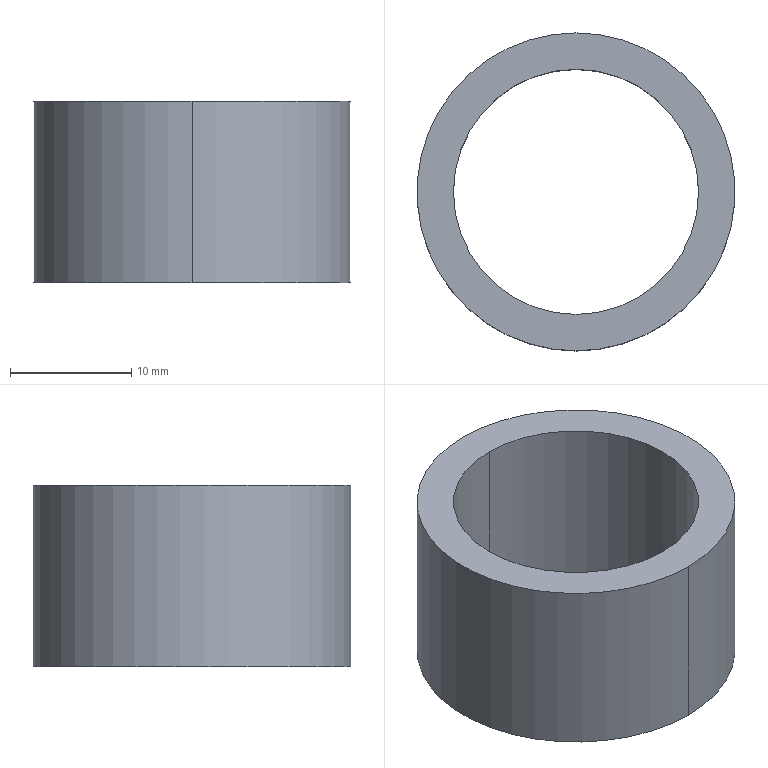Component | SolidWorks | TractionDriveWheelAssembly-1_TractionDriveWheelLimitSleeve3-1 | 1 solid | 6 faces | box 26.2 x 26.2 x 15 mm | volume 3280 mm3 | cylinder 4 | plane 2 | commonest cylinder face diameters 20.2 x2 26.2 x2
build123d program:
from build123d import *

# Parameters (mm, degrees)
SKETCH1_R           = 13.1
SKETCH1_R_2         = 10.1
BOSS_EXTRUDE1_DEPTH = 15


with BuildPart() as part:
    # Sketch1 → Boss-Extrude1 (new body)
    with BuildSketch(Plane.XY):
        Circle(SKETCH1_R)
        Circle(SKETCH1_R_2, mode=Mode.SUBTRACT)
    extrude(amount=BOSS_EXTRUDE1_DEPTH)


solid = part.part

# Placed as in the assembly
solid = solid.moved(Location((-299.507, -39.911, 395), (0, 0, 0)))
STEP:
#1=COLOUR_RGB('',0.7922,0.8196,0.9333);
#2=FILL_AREA_STYLE_COLOUR('',#1);
#3=FILL_AREA_STYLE('',(#2));
#4=SURFACE_STYLE_FILL_AREA(#3);
#5=SURFACE_SIDE_STYLE('',(#4));
#6=SURFACE_STYLE_USAGE(.BOTH.,#5);
#7=PRESENTATION_STYLE_ASSIGNMENT((#6));
#8=CARTESIAN_POINT('',(-11.792,-1.969,16.142));
#9=VERTEX_POINT('',#8);
#10=CARTESIAN_POINT('',(-11.792,-1.174,16.142));
#11=VERTEX_POINT('',#10);
#12=CARTESIAN_POINT('',(-11.792,-1.571,16.142));
#13=DIRECTION('',(-0.,-0.,1.));
#14=DIRECTION('',(-0.,1.,0.));
#15=AXIS2_PLACEMENT_3D('',#12,#13,#14);
#16=CIRCLE('',#15,0.3976);
#17=EDGE_CURVE('',#9,#11,#16,.T.);
#18=ORIENTED_EDGE('',*,*,#17,.T.);
#19=CARTESIAN_POINT('',(-11.792,-1.174,15.551));
#20=VERTEX_POINT('',#19);
#21=CARTESIAN_POINT('',(-11.792,-1.174,16.142));
#22=DIRECTION('',(0.,0.,-1.));
#23=VECTOR('',#22,39.37);
#24=LINE('',#21,#23);
#25=EDGE_CURVE('',#11,#20,#24,.T.);
#26=ORIENTED_EDGE('',*,*,#25,.T.);
#27=CARTESIAN_POINT('',(-11.792,-1.969,15.551));
#28=VERTEX_POINT('',#27);
#29=CARTESIAN_POINT('',(-11.792,-1.571,15.551));
#30=DIRECTION('',(-0.,-0.,1.));
#31=DIRECTION('',(-0.,1.,0.));
#32=AXIS2_PLACEMENT_3D('',#29,#30,#31);
#33=CIRCLE('',#32,0.3976);
#34=EDGE_CURVE('',#28,#20,#33,.T.);
#35=ORIENTED_EDGE('',*,*,#34,.F.);
#36=CARTESIAN_POINT('',(-11.792,-1.969,16.142));
#37=DIRECTION('',(0.,0.,-1.));
#38=VECTOR('',#37,39.37);
#39=LINE('',#36,#38);
#40=EDGE_CURVE('',#9,#28,#39,.T.);
#41=ORIENTED_EDGE('',*,*,#40,.F.);
#42=EDGE_LOOP('',(#18,#26,#35,#41));
#43=FACE_OUTER_BOUND('',#42,.T.);
#44=CARTESIAN_POINT('',(-11.792,-1.571,16.142));
#45=DIRECTION('',(0.,0.,-1.));
#46=DIRECTION('',(0.,-1.,0.));
#47=AXIS2_PLACEMENT_3D('',#44,#45,#46);
#48=CYLINDRICAL_SURFACE('',#47,0.3976);
#49=ADVANCED_FACE('',(#43),#48,.F.);
#50=CARTESIAN_POINT('',(-11.792,-1.056,16.142));
#51=VERTEX_POINT('',#50);
#52=CARTESIAN_POINT('',(-11.792,-2.087,16.142));
#53=VERTEX_POINT('',#52);
#54=CARTESIAN_POINT('',(-11.792,-1.571,16.142));
#55=DIRECTION('',(-0.,-0.,1.));
#56=DIRECTION('',(-0.,1.,0.));
#57=AXIS2_PLACEMENT_3D('',#54,#55,#56);
#58=CIRCLE('',#57,0.5157);
#59=EDGE_CURVE('',#51,#53,#58,.T.);
#60=ORIENTED_EDGE('',*,*,#59,.F.);
#61=CARTESIAN_POINT('',(-11.792,-1.056,15.551));
#62=VERTEX_POINT('',#61);
#63=CARTESIAN_POINT('',(-11.792,-1.056,16.142));
#64=DIRECTION('',(0.,0.,-1.));
#65=VECTOR('',#64,39.37);
#66=LINE('',#63,#65);
#67=EDGE_CURVE('',#51,#62,#66,.T.);
#68=ORIENTED_EDGE('',*,*,#67,.T.);
#69=CARTESIAN_POINT('',(-11.792,-2.087,15.551));
#70=VERTEX_POINT('',#69);
#71=CARTESIAN_POINT('',(-11.792,-1.571,15.551));
#72=DIRECTION('',(-0.,-0.,1.));
#73=DIRECTION('',(-0.,1.,0.));
#74=AXIS2_PLACEMENT_3D('',#71,#72,#73);
#75=CIRCLE('',#74,0.5157);
#76=EDGE_CURVE('',#62,#70,#75,.T.);
#77=ORIENTED_EDGE('',*,*,#76,.T.);
#78=CARTESIAN_POINT('',(-11.792,-2.087,16.142));
#79=DIRECTION('',(0.,0.,-1.));
#80=VECTOR('',#79,39.37);
#81=LINE('',#78,#80);
#82=EDGE_CURVE('',#53,#70,#81,.T.);
#83=ORIENTED_EDGE('',*,*,#82,.F.);
#84=EDGE_LOOP('',(#60,#68,#77,#83));
#85=FACE_OUTER_BOUND('',#84,.T.);
#86=CARTESIAN_POINT('',(-11.792,-1.571,16.142));
#87=DIRECTION('',(0.,0.,-1.));
#88=DIRECTION('',(0.,-1.,0.));
#89=AXIS2_PLACEMENT_3D('',#86,#87,#88);
#90=CYLINDRICAL_SURFACE('',#89,0.5157);
#91=ADVANCED_FACE('',(#85),#90,.T.);
#92=CARTESIAN_POINT('',(-11.792,-1.571,16.142));
#93=DIRECTION('',(-0.,-0.,1.));
#94=DIRECTION('',(-0.,1.,0.));
#95=AXIS2_PLACEMENT_3D('',#92,#93,#94);
#96=CIRCLE('',#95,0.5157);
#97=EDGE_CURVE('',#53,#51,#96,.T.);
#98=ORIENTED_EDGE('',*,*,#97,.T.);
#99=ORIENTED_EDGE('',*,*,#59,.T.);
#100=EDGE_LOOP('',(#98,#99));
#101=FACE_OUTER_BOUND('',#100,.T.);
#102=ORIENTED_EDGE('',*,*,#17,.F.);
#103=CARTESIAN_POINT('',(-11.792,-1.571,16.142));
#104=DIRECTION('',(-0.,-0.,1.));
#105=DIRECTION('',(-0.,1.,0.));
#106=AXIS2_PLACEMENT_3D('',#103,#104,#105);
#107=CIRCLE('',#106,0.3976);
#108=EDGE_CURVE('',#11,#9,#107,.T.);
#109=ORIENTED_EDGE('',*,*,#108,.F.);
#110=EDGE_LOOP('',(#102,#109));
#111=FACE_BOUND('',#110,.T.);
#112=CARTESIAN_POINT('',(-11.792,-1.571,16.142));
#113=DIRECTION('',(-0.,-0.,1.));
#114=DIRECTION('',(-0.,1.,0.));
#115=AXIS2_PLACEMENT_3D('',#112,#113,#114);
#116=PLANE('',#115);
#117=ADVANCED_FACE('',(#101,#111),#116,.T.);
#118=CARTESIAN_POINT('',(-11.792,-1.571,15.551));
#119=DIRECTION('',(-0.,-0.,1.));
#120=DIRECTION('',(-0.,1.,0.));
#121=AXIS2_PLACEMENT_3D('',#118,#119,#120);
#122=CIRCLE('',#121,0.5157);
#123=EDGE_CURVE('',#70,#62,#122,.T.);
#124=ORIENTED_EDGE('',*,*,#123,.F.);
#125=ORIENTED_EDGE('',*,*,#76,.F.);
#126=EDGE_LOOP('',(#124,#125));
#127=FACE_OUTER_BOUND('',#126,.T.);
#128=ORIENTED_EDGE('',*,*,#34,.T.);
#129=CARTESIAN_POINT('',(-11.792,-1.571,15.551));
#130=DIRECTION('',(-0.,-0.,1.));
#131=DIRECTION('',(-0.,1.,0.));
#132=AXIS2_PLACEMENT_3D('',#129,#130,#131);
#133=CIRCLE('',#132,0.3976);
#134=EDGE_CURVE('',#20,#28,#133,.T.);
#135=ORIENTED_EDGE('',*,*,#134,.T.);
#136=EDGE_LOOP('',(#128,#135));
#137=FACE_BOUND('',#136,.T.);
#138=CARTESIAN_POINT('',(-11.792,-1.571,15.551));
#139=DIRECTION('',(-0.,-0.,1.));
#140=DIRECTION('',(-0.,1.,0.));
#141=AXIS2_PLACEMENT_3D('',#138,#139,#140);
#142=PLANE('',#141);
#143=ADVANCED_FACE('',(#127,#137),#142,.F.);
#144=ORIENTED_EDGE('',*,*,#67,.F.);
#145=ORIENTED_EDGE('',*,*,#97,.F.);
#146=ORIENTED_EDGE('',*,*,#82,.T.);
#147=ORIENTED_EDGE('',*,*,#123,.T.);
#148=EDGE_LOOP('',(#144,#145,#146,#147));
#149=FACE_OUTER_BOUND('',#148,.T.);
#150=CARTESIAN_POINT('',(-11.792,-1.571,16.142));
#151=DIRECTION('',(0.,0.,-1.));
#152=DIRECTION('',(0.,-1.,0.));
#153=AXIS2_PLACEMENT_3D('',#150,#151,#152);
#154=CYLINDRICAL_SURFACE('',#153,0.5157);
#155=ADVANCED_FACE('',(#149),#154,.T.);
#156=ORIENTED_EDGE('',*,*,#25,.F.);
#157=ORIENTED_EDGE('',*,*,#108,.T.);
#158=ORIENTED_EDGE('',*,*,#40,.T.);
#159=ORIENTED_EDGE('',*,*,#134,.F.);
#160=EDGE_LOOP('',(#156,#157,#158,#159));
#161=FACE_OUTER_BOUND('',#160,.T.);
#162=CARTESIAN_POINT('',(-11.792,-1.571,16.142));
#163=DIRECTION('',(0.,0.,-1.));
#164=DIRECTION('',(0.,-1.,0.));
#165=AXIS2_PLACEMENT_3D('',#162,#163,#164);
#166=CYLINDRICAL_SURFACE('',#165,0.3976);
#167=ADVANCED_FACE('',(#161),#166,.F.);
#168=CLOSED_SHELL('',(#49,#91,#117,#143,#155,#167));
#169=MANIFOLD_SOLID_BREP('',#168);
#170=STYLED_ITEM('',(#7),#169);
#171=PRESENTATION_LAYER_ASSIGNMENT('','',(#170));
#172=(LENGTH_UNIT()NAMED_UNIT(*)SI_UNIT($,.METRE.));
#173=LENGTH_MEASURE_WITH_UNIT(LENGTH_MEASURE(0.0254),#172);
#174=DIMENSIONAL_EXPONENTS(1.,0.,0.,0.,0.,0.,0.);
#175=(CONVERSION_BASED_UNIT('',#173)LENGTH_UNIT()NAMED_UNIT(#174));
#176=UNCERTAINTY_MEASURE_WITH_UNIT(LENGTH_MEASURE(0.00001),#175,'','');
#177=(NAMED_UNIT(*)PLANE_ANGLE_UNIT()SI_UNIT($,.RADIAN.));
#178=(NAMED_UNIT(*)SI_UNIT($,.STERADIAN.)SOLID_ANGLE_UNIT());
#179=(GEOMETRIC_REPRESENTATION_CONTEXT(3)GLOBAL_UNCERTAINTY_ASSIGNED_CONTEXT((#176))GLOBAL_UNIT_ASSIGNED_CONTEXT((#175,#177,#178))REPRESENTATION_CONTEXT('',''));
#180=MECHANICAL_DESIGN_GEOMETRIC_PRESENTATION_REPRESENTATION('',(#170),#179);
#181=CARTESIAN_POINT('',(0.,0.,0.));
#182=DIRECTION('',(0.,0.,1.));
#183=DIRECTION('',(1.,0.,0.));
#184=AXIS2_PLACEMENT_3D('',#181,#182,#183);
#185=(LENGTH_UNIT()NAMED_UNIT(*)SI_UNIT($,.METRE.));
#186=LENGTH_MEASURE_WITH_UNIT(LENGTH_MEASURE(0.0254),#185);
#187=DIMENSIONAL_EXPONENTS(1.,0.,0.,0.,0.,0.,0.);
#188=(CONVERSION_BASED_UNIT('',#186)LENGTH_UNIT()NAMED_UNIT(#187));
#189=UNCERTAINTY_MEASURE_WITH_UNIT(LENGTH_MEASURE(0.00001),#188,'','');
#190=(NAMED_UNIT(*)PLANE_ANGLE_UNIT()SI_UNIT($,.RADIAN.));
#191=(NAMED_UNIT(*)SI_UNIT($,.STERADIAN.)SOLID_ANGLE_UNIT());
#192=(GEOMETRIC_REPRESENTATION_CONTEXT(3)GLOBAL_UNCERTAINTY_ASSIGNED_CONTEXT((#189))GLOBAL_UNIT_ASSIGNED_CONTEXT((#188,#190,#191))REPRESENTATION_CONTEXT('',''));
#193=ADVANCED_BREP_SHAPE_REPRESENTATION('',(#169,#184),#192);